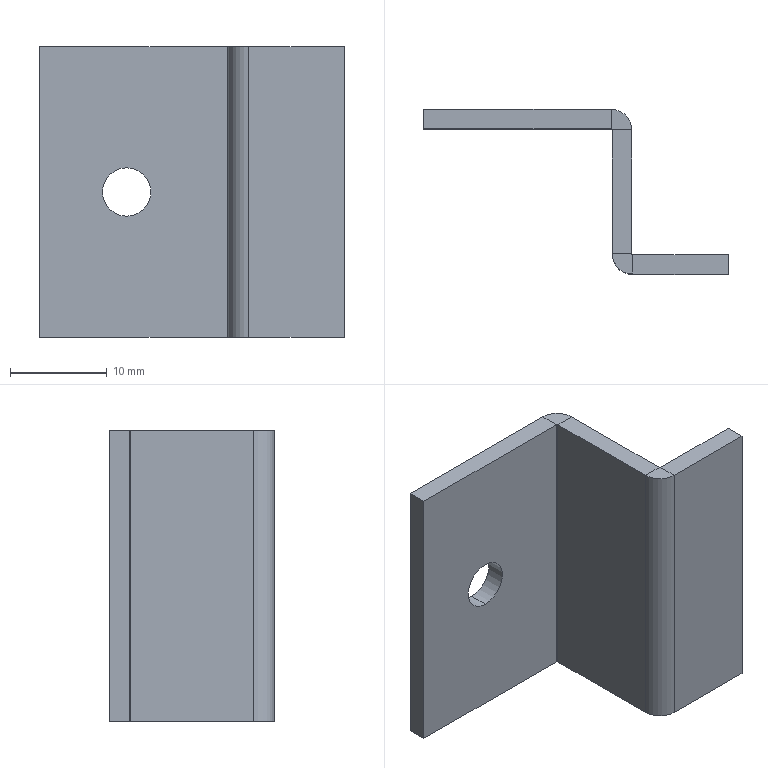Component | SolidWorks | FrontDoorAssembly-1_GlassRetainerPG50-02-105-10 | 1 solid | 24 faces | box 31.5 x 17 x 30 mm | volume 2694 mm3 | plane 18 | cylinder 6 | commonest cylinder face diameters 5 x2 4.2 x2 0.2 x2 | material AISI 1045 Steel, cold drawn
STEP:
#1=COLOUR_RGB('',0.7922,0.8196,0.9333);
#2=FILL_AREA_STYLE_COLOUR('',#1);
#3=FILL_AREA_STYLE('',(#2));
#4=SURFACE_STYLE_FILL_AREA(#3);
#5=SURFACE_SIDE_STYLE('',(#4));
#6=SURFACE_STYLE_USAGE(.BOTH.,#5);
#7=PRESENTATION_STYLE_ASSIGNMENT((#6));
#8=CARTESIAN_POINT('',(-43.629,-10.307,10.729));
#9=VERTEX_POINT('',#8);
#10=CARTESIAN_POINT('',(-43.629,-10.307,10.925));
#11=VERTEX_POINT('',#10);
#12=CARTESIAN_POINT('',(-43.629,-10.307,10.827));
#13=DIRECTION('',(-0.,1.,0.));
#14=DIRECTION('',(0.,0.,1.));
#15=AXIS2_PLACEMENT_3D('',#12,#13,#14);
#16=CIRCLE('',#15,0.09843);
#17=EDGE_CURVE('',#9,#11,#16,.T.);
#18=ORIENTED_EDGE('',*,*,#17,.F.);
#19=CARTESIAN_POINT('',(-43.629,-10.228,10.729));
#20=VERTEX_POINT('',#19);
#21=CARTESIAN_POINT('',(-43.629,-10.228,10.729));
#22=DIRECTION('',(-0.,1.,0.));
#23=VECTOR('',#22,39.37);
#24=LINE('',#21,#23);
#25=EDGE_CURVE('',#9,#20,#24,.T.);
#26=ORIENTED_EDGE('',*,*,#25,.T.);
#27=CARTESIAN_POINT('',(-43.629,-10.228,10.925));
#28=VERTEX_POINT('',#27);
#29=CARTESIAN_POINT('',(-43.629,-10.228,10.827));
#30=DIRECTION('',(-0.,1.,0.));
#31=DIRECTION('',(0.,0.,1.));
#32=AXIS2_PLACEMENT_3D('',#29,#30,#31);
#33=CIRCLE('',#32,0.09843);
#34=EDGE_CURVE('',#20,#28,#33,.T.);
#35=ORIENTED_EDGE('',*,*,#34,.T.);
#36=CARTESIAN_POINT('',(-43.629,-10.228,10.925));
#37=DIRECTION('',(-0.,1.,0.));
#38=VECTOR('',#37,39.37);
#39=LINE('',#36,#38);
#40=EDGE_CURVE('',#11,#28,#39,.T.);
#41=ORIENTED_EDGE('',*,*,#40,.F.);
#42=EDGE_LOOP('',(#18,#26,#35,#41));
#43=FACE_OUTER_BOUND('',#42,.T.);
#44=CARTESIAN_POINT('',(-43.629,-10.228,10.827));
#45=DIRECTION('',(-0.,1.,0.));
#46=DIRECTION('',(0.,0.,1.));
#47=AXIS2_PLACEMENT_3D('',#44,#45,#46);
#48=CYLINDRICAL_SURFACE('',#47,0.09843);
#49=ADVANCED_FACE('',(#43),#48,.F.);
#50=CARTESIAN_POINT('',(-43.216,-10.815,10.236));
#51=VERTEX_POINT('',#50);
#52=CARTESIAN_POINT('',(-43.137,-10.815,10.236));
#53=VERTEX_POINT('',#52);
#54=CARTESIAN_POINT('',(-43.137,-10.815,10.236));
#55=DIRECTION('',(1.,0.,0.));
#56=VECTOR('',#55,39.37);
#57=LINE('',#54,#56);
#58=EDGE_CURVE('',#51,#53,#57,.T.);
#59=ORIENTED_EDGE('',*,*,#58,.F.);
#60=CARTESIAN_POINT('',(-43.216,-10.311,10.236));
#61=VERTEX_POINT('',#60);
#62=CARTESIAN_POINT('',(-43.216,-10.819,10.236));
#63=DIRECTION('',(0.,-1.,-0.));
#64=VECTOR('',#63,39.37);
#65=LINE('',#62,#64);
#66=EDGE_CURVE('',#61,#51,#65,.T.);
#67=ORIENTED_EDGE('',*,*,#66,.F.);
#68=CARTESIAN_POINT('',(-43.137,-10.311,10.236));
#69=VERTEX_POINT('',#68);
#70=CARTESIAN_POINT('',(-43.137,-10.311,10.236));
#71=DIRECTION('',(1.,0.,0.));
#72=VECTOR('',#71,39.37);
#73=LINE('',#70,#72);
#74=EDGE_CURVE('',#61,#69,#73,.T.);
#75=ORIENTED_EDGE('',*,*,#74,.T.);
#76=CARTESIAN_POINT('',(-43.137,-10.819,10.236));
#77=DIRECTION('',(0.,-1.,-0.));
#78=VECTOR('',#77,39.37);
#79=LINE('',#76,#78);
#80=EDGE_CURVE('',#69,#53,#79,.T.);
#81=ORIENTED_EDGE('',*,*,#80,.T.);
#82=EDGE_LOOP('',(#59,#67,#75,#81));
#83=FACE_OUTER_BOUND('',#82,.T.);
#84=CARTESIAN_POINT('',(-43.137,-10.819,10.236));
#85=DIRECTION('',(0.,0.,-1.));
#86=DIRECTION('',(0.,-1.,-0.));
#87=AXIS2_PLACEMENT_3D('',#84,#85,#86);
#88=PLANE('',#87);
#89=ADVANCED_FACE('',(#83),#88,.T.);
#90=ORIENTED_EDGE('',*,*,#74,.F.);
#91=CARTESIAN_POINT('',(-43.22,-10.307,10.236));
#92=VERTEX_POINT('',#91);
#93=CARTESIAN_POINT('',(-43.22,-10.311,10.236));
#94=DIRECTION('',(-0.,-0.,1.));
#95=DIRECTION('',(0.,-1.,0.));
#96=AXIS2_PLACEMENT_3D('',#93,#94,#95);
#97=CIRCLE('',#96,0.003937);
#98=EDGE_CURVE('',#61,#92,#97,.T.);
#99=ORIENTED_EDGE('',*,*,#98,.T.);
#100=CARTESIAN_POINT('',(-43.22,-10.228,10.236));
#101=VERTEX_POINT('',#100);
#102=CARTESIAN_POINT('',(-43.22,-10.228,10.236));
#103=DIRECTION('',(-0.,1.,0.));
#104=VECTOR('',#103,39.37);
#105=LINE('',#102,#104);
#106=EDGE_CURVE('',#92,#101,#105,.T.);
#107=ORIENTED_EDGE('',*,*,#106,.T.);
#108=CARTESIAN_POINT('',(-43.22,-10.311,10.236));
#109=DIRECTION('',(-0.,-0.,1.));
#110=DIRECTION('',(0.,1.,0.));
#111=AXIS2_PLACEMENT_3D('',#108,#109,#110);
#112=CIRCLE('',#111,0.08268);
#113=EDGE_CURVE('',#69,#101,#112,.T.);
#114=ORIENTED_EDGE('',*,*,#113,.F.);
#115=EDGE_LOOP('',(#90,#99,#107,#114));
#116=FACE_OUTER_BOUND('',#115,.T.);
#117=CARTESIAN_POINT('',(-43.22,-10.311,10.236));
#118=DIRECTION('',(-0.,-0.,1.));
#119=DIRECTION('',(0.,-1.,-0.));
#120=AXIS2_PLACEMENT_3D('',#117,#118,#119);
#121=PLANE('',#120);
#122=ADVANCED_FACE('',(#116),#121,.F.);
#123=ORIENTED_EDGE('',*,*,#106,.F.);
#124=CARTESIAN_POINT('',(-43.984,-10.307,10.236));
#125=VERTEX_POINT('',#124);
#126=CARTESIAN_POINT('',(-43.137,-10.307,10.236));
#127=DIRECTION('',(1.,0.,0.));
#128=VECTOR('',#127,39.37);
#129=LINE('',#126,#128);
#130=EDGE_CURVE('',#125,#92,#129,.T.);
#131=ORIENTED_EDGE('',*,*,#130,.F.);
#132=CARTESIAN_POINT('',(-43.984,-10.228,10.236));
#133=VERTEX_POINT('',#132);
#134=CARTESIAN_POINT('',(-43.984,-10.228,10.236));
#135=DIRECTION('',(-0.,1.,0.));
#136=VECTOR('',#135,39.37);
#137=LINE('',#134,#136);
#138=EDGE_CURVE('',#125,#133,#137,.T.);
#139=ORIENTED_EDGE('',*,*,#138,.T.);
#140=CARTESIAN_POINT('',(-43.137,-10.228,10.236));
#141=DIRECTION('',(1.,0.,0.));
#142=VECTOR('',#141,39.37);
#143=LINE('',#140,#142);
#144=EDGE_CURVE('',#133,#101,#143,.T.);
#145=ORIENTED_EDGE('',*,*,#144,.T.);
#146=EDGE_LOOP('',(#123,#131,#139,#145));
#147=FACE_OUTER_BOUND('',#146,.T.);
#148=CARTESIAN_POINT('',(-43.137,-10.228,10.236));
#149=DIRECTION('',(0.,0.,-1.));
#150=DIRECTION('',(1.,0.,0.));
#151=AXIS2_PLACEMENT_3D('',#148,#149,#150);
#152=PLANE('',#151);
#153=ADVANCED_FACE('',(#147),#152,.T.);
#154=ORIENTED_EDGE('',*,*,#138,.F.);
#155=CARTESIAN_POINT('',(-43.984,-10.307,11.417));
#156=VERTEX_POINT('',#155);
#157=CARTESIAN_POINT('',(-43.984,-10.307,10.236));
#158=DIRECTION('',(-0.,-0.,1.));
#159=VECTOR('',#158,39.37);
#160=LINE('',#157,#159);
#161=EDGE_CURVE('',#125,#156,#160,.T.);
#162=ORIENTED_EDGE('',*,*,#161,.T.);
#163=CARTESIAN_POINT('',(-43.984,-10.228,11.417));
#164=VERTEX_POINT('',#163);
#165=CARTESIAN_POINT('',(-43.984,-10.228,11.417));
#166=DIRECTION('',(-0.,1.,0.));
#167=VECTOR('',#166,39.37);
#168=LINE('',#165,#167);
#169=EDGE_CURVE('',#156,#164,#168,.T.);
#170=ORIENTED_EDGE('',*,*,#169,.T.);
#171=CARTESIAN_POINT('',(-43.984,-10.228,10.236));
#172=DIRECTION('',(-0.,-0.,1.));
#173=VECTOR('',#172,39.37);
#174=LINE('',#171,#173);
#175=EDGE_CURVE('',#133,#164,#174,.T.);
#176=ORIENTED_EDGE('',*,*,#175,.F.);
#177=EDGE_LOOP('',(#154,#162,#170,#176));
#178=FACE_OUTER_BOUND('',#177,.T.);
#179=CARTESIAN_POINT('',(-43.984,-10.228,10.236));
#180=DIRECTION('',(1.,0.,0.));
#181=DIRECTION('',(-0.,-0.,1.));
#182=AXIS2_PLACEMENT_3D('',#179,#180,#181);
#183=PLANE('',#182);
#184=ADVANCED_FACE('',(#178),#183,.F.);
#185=ORIENTED_EDGE('',*,*,#169,.F.);
#186=CARTESIAN_POINT('',(-43.22,-10.307,11.417));
#187=VERTEX_POINT('',#186);
#188=CARTESIAN_POINT('',(-43.137,-10.307,11.417));
#189=DIRECTION('',(1.,0.,0.));
#190=VECTOR('',#189,39.37);
#191=LINE('',#188,#190);
#192=EDGE_CURVE('',#156,#187,#191,.T.);
#193=ORIENTED_EDGE('',*,*,#192,.T.);
#194=CARTESIAN_POINT('',(-43.22,-10.228,11.417));
#195=VERTEX_POINT('',#194);
#196=CARTESIAN_POINT('',(-43.22,-10.228,11.417));
#197=DIRECTION('',(-0.,1.,0.));
#198=VECTOR('',#197,39.37);
#199=LINE('',#196,#198);
#200=EDGE_CURVE('',#187,#195,#199,.T.);
#201=ORIENTED_EDGE('',*,*,#200,.T.);
#202=CARTESIAN_POINT('',(-43.137,-10.228,11.417));
#203=DIRECTION('',(1.,0.,0.));
#204=VECTOR('',#203,39.37);
#205=LINE('',#202,#204);
#206=EDGE_CURVE('',#164,#195,#205,.T.);
#207=ORIENTED_EDGE('',*,*,#206,.F.);
#208=EDGE_LOOP('',(#185,#193,#201,#207));
#209=FACE_OUTER_BOUND('',#208,.T.);
#210=CARTESIAN_POINT('',(-43.137,-10.228,11.417));
#211=DIRECTION('',(0.,0.,-1.));
#212=DIRECTION('',(1.,0.,0.));
#213=AXIS2_PLACEMENT_3D('',#210,#211,#212);
#214=PLANE('',#213);
#215=ADVANCED_FACE('',(#209),#214,.F.);
#216=ORIENTED_EDGE('',*,*,#200,.F.);
#217=CARTESIAN_POINT('',(-43.216,-10.311,11.417));
#218=VERTEX_POINT('',#217);
#219=CARTESIAN_POINT('',(-43.22,-10.311,11.417));
#220=DIRECTION('',(0.,0.,-1.));
#221=DIRECTION('',(0.,-1.,0.));
#222=AXIS2_PLACEMENT_3D('',#219,#220,#221);
#223=CIRCLE('',#222,0.003937);
#224=EDGE_CURVE('',#187,#218,#223,.T.);
#225=ORIENTED_EDGE('',*,*,#224,.T.);
#226=CARTESIAN_POINT('',(-43.137,-10.311,11.417));
#227=VERTEX_POINT('',#226);
#228=CARTESIAN_POINT('',(-43.137,-10.311,11.417));
#229=DIRECTION('',(1.,0.,0.));
#230=VECTOR('',#229,39.37);
#231=LINE('',#228,#230);
#232=EDGE_CURVE('',#218,#227,#231,.T.);
#233=ORIENTED_EDGE('',*,*,#232,.T.);
#234=CARTESIAN_POINT('',(-43.22,-10.311,11.417));
#235=DIRECTION('',(0.,0.,-1.));
#236=DIRECTION('',(0.,-1.,0.));
#237=AXIS2_PLACEMENT_3D('',#234,#235,#236);
#238=CIRCLE('',#237,0.08268);
#239=EDGE_CURVE('',#195,#227,#238,.T.);
#240=ORIENTED_EDGE('',*,*,#239,.F.);
#241=EDGE_LOOP('',(#216,#225,#233,#240));
#242=FACE_OUTER_BOUND('',#241,.T.);
#243=CARTESIAN_POINT('',(-43.22,-10.311,11.417));
#244=DIRECTION('',(0.,0.,-1.));
#245=DIRECTION('',(-0.,1.,0.));
#246=AXIS2_PLACEMENT_3D('',#243,#244,#245);
#247=PLANE('',#246);
#248=ADVANCED_FACE('',(#242),#247,.F.);
#249=ORIENTED_EDGE('',*,*,#232,.F.);
#250=CARTESIAN_POINT('',(-43.216,-10.815,11.417));
#251=VERTEX_POINT('',#250);
#252=CARTESIAN_POINT('',(-43.216,-10.819,11.417));
#253=DIRECTION('',(0.,-1.,-0.));
#254=VECTOR('',#253,39.37);
#255=LINE('',#252,#254);
#256=EDGE_CURVE('',#218,#251,#255,.T.);
#257=ORIENTED_EDGE('',*,*,#256,.T.);
#258=CARTESIAN_POINT('',(-43.137,-10.815,11.417));
#259=VERTEX_POINT('',#258);
#260=CARTESIAN_POINT('',(-43.137,-10.815,11.417));
#261=DIRECTION('',(1.,0.,0.));
#262=VECTOR('',#261,39.37);
#263=LINE('',#260,#262);
#264=EDGE_CURVE('',#251,#259,#263,.T.);
#265=ORIENTED_EDGE('',*,*,#264,.T.);
#266=CARTESIAN_POINT('',(-43.137,-10.819,11.417));
#267=DIRECTION('',(0.,-1.,-0.));
#268=VECTOR('',#267,39.37);
#269=LINE('',#266,#268);
#270=EDGE_CURVE('',#227,#259,#269,.T.);
#271=ORIENTED_EDGE('',*,*,#270,.F.);
#272=EDGE_LOOP('',(#249,#257,#265,#271));
#273=FACE_OUTER_BOUND('',#272,.T.);
#274=CARTESIAN_POINT('',(-43.137,-10.819,11.417));
#275=DIRECTION('',(0.,0.,-1.));
#276=DIRECTION('',(0.,-1.,-0.));
#277=AXIS2_PLACEMENT_3D('',#274,#275,#276);
#278=PLANE('',#277);
#279=ADVANCED_FACE('',(#273),#278,.F.);
#280=ORIENTED_EDGE('',*,*,#264,.F.);
#281=CARTESIAN_POINT('',(-43.133,-10.898,11.417));
#282=VERTEX_POINT('',#281);
#283=CARTESIAN_POINT('',(-43.133,-10.815,11.417));
#284=DIRECTION('',(-0.,-0.,1.));
#285=DIRECTION('',(0.,1.,0.));
#286=AXIS2_PLACEMENT_3D('',#283,#284,#285);
#287=CIRCLE('',#286,0.08268);
#288=EDGE_CURVE('',#251,#282,#287,.T.);
#289=ORIENTED_EDGE('',*,*,#288,.T.);
#290=CARTESIAN_POINT('',(-43.133,-10.819,11.417));
#291=VERTEX_POINT('',#290);
#292=CARTESIAN_POINT('',(-43.133,-10.819,11.417));
#293=DIRECTION('',(-0.,1.,0.));
#294=VECTOR('',#293,39.37);
#295=LINE('',#292,#294);
#296=EDGE_CURVE('',#282,#291,#295,.T.);
#297=ORIENTED_EDGE('',*,*,#296,.T.);
#298=CARTESIAN_POINT('',(-43.133,-10.815,11.417));
#299=DIRECTION('',(-0.,-0.,1.));
#300=DIRECTION('',(0.,1.,0.));
#301=AXIS2_PLACEMENT_3D('',#298,#299,#300);
#302=CIRCLE('',#301,0.003937);
#303=EDGE_CURVE('',#259,#291,#302,.T.);
#304=ORIENTED_EDGE('',*,*,#303,.F.);
#305=EDGE_LOOP('',(#280,#289,#297,#304));
#306=FACE_OUTER_BOUND('',#305,.T.);
#307=CARTESIAN_POINT('',(-43.133,-10.815,11.417));
#308=DIRECTION('',(-0.,-0.,1.));
#309=DIRECTION('',(0.,-1.,-0.));
#310=AXIS2_PLACEMENT_3D('',#307,#308,#309);
#311=PLANE('',#310);
#312=ADVANCED_FACE('',(#306),#311,.T.);
#313=CARTESIAN_POINT('',(-42.744,-10.898,11.417));
#314=VERTEX_POINT('',#313);
#315=CARTESIAN_POINT('',(-42.744,-10.819,11.417));
#316=VERTEX_POINT('',#315);
#317=CARTESIAN_POINT('',(-42.744,-11.213,11.417));
#318=DIRECTION('',(-0.,1.,0.));
#319=VECTOR('',#318,39.37);
#320=LINE('',#317,#319);
#321=EDGE_CURVE('',#314,#316,#320,.T.);
#322=ORIENTED_EDGE('',*,*,#321,.T.);
#323=CARTESIAN_POINT('',(-42.629,-10.819,11.417));
#324=DIRECTION('',(1.,0.,0.));
#325=VECTOR('',#324,39.37);
#326=LINE('',#323,#325);
#327=EDGE_CURVE('',#291,#316,#326,.T.);
#328=ORIENTED_EDGE('',*,*,#327,.F.);
#329=ORIENTED_EDGE('',*,*,#296,.F.);
#330=CARTESIAN_POINT('',(-42.629,-10.898,11.417));
#331=DIRECTION('',(1.,0.,0.));
#332=VECTOR('',#331,39.37);
#333=LINE('',#330,#332);
#334=EDGE_CURVE('',#282,#314,#333,.T.);
#335=ORIENTED_EDGE('',*,*,#334,.T.);
#336=EDGE_LOOP('',(#322,#328,#329,#335));
#337=FACE_OUTER_BOUND('',#336,.T.);
#338=CARTESIAN_POINT('',(-42.629,-10.819,11.417));
#339=DIRECTION('',(0.,0.,-1.));
#340=DIRECTION('',(1.,0.,0.));
#341=AXIS2_PLACEMENT_3D('',#338,#339,#340);
#342=PLANE('',#341);
#343=ADVANCED_FACE('',(#337),#342,.F.);
#344=CARTESIAN_POINT('',(-42.744,-10.898,10.236));
#345=VERTEX_POINT('',#344);
#346=CARTESIAN_POINT('',(-42.744,-10.819,10.236));
#347=VERTEX_POINT('',#346);
#348=CARTESIAN_POINT('',(-42.744,-11.213,10.236));
#349=DIRECTION('',(-0.,1.,0.));
#350=VECTOR('',#349,39.37);
#351=LINE('',#348,#350);
#352=EDGE_CURVE('',#345,#347,#351,.T.);
#353=ORIENTED_EDGE('',*,*,#352,.F.);
#354=CARTESIAN_POINT('',(-43.133,-10.898,10.236));
#355=VERTEX_POINT('',#354);
#356=CARTESIAN_POINT('',(-42.629,-10.898,10.236));
#357=DIRECTION('',(1.,0.,0.));
#358=VECTOR('',#357,39.37);
#359=LINE('',#356,#358);
#360=EDGE_CURVE('',#355,#345,#359,.T.);
#361=ORIENTED_EDGE('',*,*,#360,.F.);
#362=CARTESIAN_POINT('',(-43.133,-10.819,10.236));
#363=VERTEX_POINT('',#362);
#364=CARTESIAN_POINT('',(-43.133,-10.819,10.236));
#365=DIRECTION('',(-0.,1.,0.));
#366=VECTOR('',#365,39.37);
#367=LINE('',#364,#366);
#368=EDGE_CURVE('',#355,#363,#367,.T.);
#369=ORIENTED_EDGE('',*,*,#368,.T.);
#370=CARTESIAN_POINT('',(-42.629,-10.819,10.236));
#371=DIRECTION('',(1.,0.,0.));
#372=VECTOR('',#371,39.37);
#373=LINE('',#370,#372);
#374=EDGE_CURVE('',#363,#347,#373,.T.);
#375=ORIENTED_EDGE('',*,*,#374,.T.);
#376=EDGE_LOOP('',(#353,#361,#369,#375));
#377=FACE_OUTER_BOUND('',#376,.T.);
#378=CARTESIAN_POINT('',(-42.629,-10.819,10.236));
#379=DIRECTION('',(0.,0.,-1.));
#380=DIRECTION('',(1.,0.,0.));
#381=AXIS2_PLACEMENT_3D('',#378,#379,#380);
#382=PLANE('',#381);
#383=ADVANCED_FACE('',(#377),#382,.T.);
#384=ORIENTED_EDGE('',*,*,#25,.F.);
#385=CARTESIAN_POINT('',(-43.629,-10.307,10.827));
#386=DIRECTION('',(-0.,1.,0.));
#387=DIRECTION('',(0.,0.,1.));
#388=AXIS2_PLACEMENT_3D('',#385,#386,#387);
#389=CIRCLE('',#388,0.09843);
#390=EDGE_CURVE('',#11,#9,#389,.T.);
#391=ORIENTED_EDGE('',*,*,#390,.F.);
#392=ORIENTED_EDGE('',*,*,#40,.T.);
#393=CARTESIAN_POINT('',(-43.629,-10.228,10.827));
#394=DIRECTION('',(-0.,1.,0.));
#395=DIRECTION('',(0.,0.,1.));
#396=AXIS2_PLACEMENT_3D('',#393,#394,#395);
#397=CIRCLE('',#396,0.09843);
#398=EDGE_CURVE('',#28,#20,#397,.T.);
#399=ORIENTED_EDGE('',*,*,#398,.T.);
#400=EDGE_LOOP('',(#384,#391,#392,#399));
#401=FACE_OUTER_BOUND('',#400,.T.);
#402=CARTESIAN_POINT('',(-43.629,-10.228,10.827));
#403=DIRECTION('',(-0.,1.,0.));
#404=DIRECTION('',(0.,0.,1.));
#405=AXIS2_PLACEMENT_3D('',#402,#403,#404);
#406=CYLINDRICAL_SURFACE('',#405,0.09843);
#407=ADVANCED_FACE('',(#401),#406,.F.);
#408=CARTESIAN_POINT('',(-43.133,-10.815,10.236));
#409=DIRECTION('',(0.,0.,-1.));
#410=DIRECTION('',(0.,1.,0.));
#411=AXIS2_PLACEMENT_3D('',#408,#409,#410);
#412=CIRCLE('',#411,0.08268);
#413=EDGE_CURVE('',#355,#51,#412,.T.);
#414=ORIENTED_EDGE('',*,*,#413,.T.);
#415=ORIENTED_EDGE('',*,*,#58,.T.);
#416=CARTESIAN_POINT('',(-43.133,-10.815,10.236));
#417=DIRECTION('',(0.,0.,-1.));
#418=DIRECTION('',(0.,-1.,0.));
#419=AXIS2_PLACEMENT_3D('',#416,#417,#418);
#420=CIRCLE('',#419,0.003937);
#421=EDGE_CURVE('',#363,#53,#420,.T.);
#422=ORIENTED_EDGE('',*,*,#421,.F.);
#423=ORIENTED_EDGE('',*,*,#368,.F.);
#424=EDGE_LOOP('',(#414,#415,#422,#423));
#425=FACE_OUTER_BOUND('',#424,.T.);
#426=CARTESIAN_POINT('',(-43.133,-10.815,10.236));
#427=DIRECTION('',(0.,0.,-1.));
#428=DIRECTION('',(-0.,1.,0.));
#429=AXIS2_PLACEMENT_3D('',#426,#427,#428);
#430=PLANE('',#429);
#431=ADVANCED_FACE('',(#425),#430,.T.);
#432=ORIENTED_EDGE('',*,*,#327,.T.);
#433=CARTESIAN_POINT('',(-42.744,-10.819,10.236));
#434=DIRECTION('',(-0.,-0.,1.));
#435=VECTOR('',#434,39.37);
#436=LINE('',#433,#435);
#437=EDGE_CURVE('',#347,#316,#436,.T.);
#438=ORIENTED_EDGE('',*,*,#437,.F.);
#439=ORIENTED_EDGE('',*,*,#374,.F.);
#440=CARTESIAN_POINT('',(-43.133,-10.819,11.417));
#441=DIRECTION('',(-0.,-0.,1.));
#442=VECTOR('',#441,39.37);
#443=LINE('',#440,#442);
#444=EDGE_CURVE('',#363,#291,#443,.T.);
#445=ORIENTED_EDGE('',*,*,#444,.T.);
#446=EDGE_LOOP('',(#432,#438,#439,#445));
#447=FACE_OUTER_BOUND('',#446,.T.);
#448=CARTESIAN_POINT('',(-42.629,-10.819,10.236));
#449=DIRECTION('',(0.,-1.,-0.));
#450=DIRECTION('',(0.,0.,-1.));
#451=AXIS2_PLACEMENT_3D('',#448,#449,#450);
#452=PLANE('',#451);
#453=ADVANCED_FACE('',(#447),#452,.F.);
#454=ORIENTED_EDGE('',*,*,#398,.F.);
#455=ORIENTED_EDGE('',*,*,#34,.F.);
#456=EDGE_LOOP('',(#454,#455));
#457=FACE_BOUND('',#456,.T.);
#458=ORIENTED_EDGE('',*,*,#206,.T.);
#459=CARTESIAN_POINT('',(-43.22,-10.228,10.236));
#460=DIRECTION('',(0.,0.,-1.));
#461=VECTOR('',#460,39.37);
#462=LINE('',#459,#461);
#463=EDGE_CURVE('',#195,#101,#462,.T.);
#464=ORIENTED_EDGE('',*,*,#463,.T.);
#465=ORIENTED_EDGE('',*,*,#144,.F.);
#466=ORIENTED_EDGE('',*,*,#175,.T.);
#467=EDGE_LOOP('',(#458,#464,#465,#466));
#468=FACE_OUTER_BOUND('',#467,.T.);
#469=CARTESIAN_POINT('',(-43.137,-10.228,10.236));
#470=DIRECTION('',(0.,-1.,-0.));
#471=DIRECTION('',(0.,0.,-1.));
#472=AXIS2_PLACEMENT_3D('',#469,#470,#471);
#473=PLANE('',#472);
#474=ADVANCED_FACE('',(#457,#468),#473,.F.);
#475=ORIENTED_EDGE('',*,*,#270,.T.);
#476=CARTESIAN_POINT('',(-43.137,-10.815,10.236));
#477=DIRECTION('',(0.,0.,-1.));
#478=VECTOR('',#477,39.37);
#479=LINE('',#476,#478);
#480=EDGE_CURVE('',#259,#53,#479,.T.);
#481=ORIENTED_EDGE('',*,*,#480,.T.);
#482=ORIENTED_EDGE('',*,*,#80,.F.);
#483=CARTESIAN_POINT('',(-43.137,-10.311,10.236));
#484=DIRECTION('',(-0.,-0.,1.));
#485=VECTOR('',#484,39.37);
#486=LINE('',#483,#485);
#487=EDGE_CURVE('',#69,#227,#486,.T.);
#488=ORIENTED_EDGE('',*,*,#487,.T.);
#489=EDGE_LOOP('',(#475,#481,#482,#488));
#490=FACE_OUTER_BOUND('',#489,.T.);
#491=CARTESIAN_POINT('',(-43.137,-10.819,10.236));
#492=DIRECTION('',(-1.,-0.,-0.));
#493=DIRECTION('',(-0.,1.,0.));
#494=AXIS2_PLACEMENT_3D('',#491,#492,#493);
#495=PLANE('',#494);
#496=ADVANCED_FACE('',(#490),#495,.F.);
#497=ORIENTED_EDGE('',*,*,#113,.T.);
#498=ORIENTED_EDGE('',*,*,#463,.F.);
#499=ORIENTED_EDGE('',*,*,#239,.T.);
#500=ORIENTED_EDGE('',*,*,#487,.F.);
#501=EDGE_LOOP('',(#497,#498,#499,#500));
#502=FACE_OUTER_BOUND('',#501,.T.);
#503=CARTESIAN_POINT('',(-43.22,-10.311,10.236));
#504=DIRECTION('',(-0.,-0.,1.));
#505=DIRECTION('',(0.,-1.,0.));
#506=AXIS2_PLACEMENT_3D('',#503,#504,#505);
#507=CYLINDRICAL_SURFACE('',#506,0.08268);
#508=ADVANCED_FACE('',(#502),#507,.T.);
#509=ORIENTED_EDGE('',*,*,#421,.T.);
#510=ORIENTED_EDGE('',*,*,#480,.F.);
#511=ORIENTED_EDGE('',*,*,#303,.T.);
#512=ORIENTED_EDGE('',*,*,#444,.F.);
#513=EDGE_LOOP('',(#509,#510,#511,#512));
#514=FACE_OUTER_BOUND('',#513,.T.);
#515=CARTESIAN_POINT('',(-43.133,-10.815,10.236));
#516=DIRECTION('',(0.,0.,-1.));
#517=DIRECTION('',(0.,1.,0.));
#518=AXIS2_PLACEMENT_3D('',#515,#516,#517);
#519=CYLINDRICAL_SURFACE('',#518,0.003937);
#520=ADVANCED_FACE('',(#514),#519,.F.);
#521=CARTESIAN_POINT('',(-42.744,-10.898,10.236));
#522=DIRECTION('',(0.,0.,-1.));
#523=VECTOR('',#522,39.37);
#524=LINE('',#521,#523);
#525=EDGE_CURVE('',#314,#345,#524,.T.);
#526=ORIENTED_EDGE('',*,*,#525,.F.);
#527=ORIENTED_EDGE('',*,*,#334,.F.);
#528=CARTESIAN_POINT('',(-43.133,-10.898,10.236));
#529=DIRECTION('',(-0.,-0.,1.));
#530=VECTOR('',#529,39.37);
#531=LINE('',#528,#530);
#532=EDGE_CURVE('',#355,#282,#531,.T.);
#533=ORIENTED_EDGE('',*,*,#532,.F.);
#534=ORIENTED_EDGE('',*,*,#360,.T.);
#535=EDGE_LOOP('',(#526,#527,#533,#534));
#536=FACE_OUTER_BOUND('',#535,.T.);
#537=CARTESIAN_POINT('',(-42.629,-10.898,10.236));
#538=DIRECTION('',(0.,-1.,-0.));
#539=DIRECTION('',(0.,0.,-1.));
#540=AXIS2_PLACEMENT_3D('',#537,#538,#539);
#541=PLANE('',#540);
#542=ADVANCED_FACE('',(#536),#541,.T.);
#543=ORIENTED_EDGE('',*,*,#390,.T.);
#544=ORIENTED_EDGE('',*,*,#17,.T.);
#545=EDGE_LOOP('',(#543,#544));
#546=FACE_BOUND('',#545,.T.);
#547=ORIENTED_EDGE('',*,*,#192,.F.);
#548=ORIENTED_EDGE('',*,*,#161,.F.);
#549=ORIENTED_EDGE('',*,*,#130,.T.);
#550=CARTESIAN_POINT('',(-43.22,-10.307,10.236));
#551=DIRECTION('',(0.,0.,-1.));
#552=VECTOR('',#551,39.37);
#553=LINE('',#550,#552);
#554=EDGE_CURVE('',#187,#92,#553,.T.);
#555=ORIENTED_EDGE('',*,*,#554,.F.);
#556=EDGE_LOOP('',(#547,#548,#549,#555));
#557=FACE_OUTER_BOUND('',#556,.T.);
#558=CARTESIAN_POINT('',(-43.137,-10.307,10.236));
#559=DIRECTION('',(0.,-1.,-0.));
#560=DIRECTION('',(0.,0.,-1.));
#561=AXIS2_PLACEMENT_3D('',#558,#559,#560);
#562=PLANE('',#561);
#563=ADVANCED_FACE('',(#546,#557),#562,.T.);
#564=ORIENTED_EDGE('',*,*,#256,.F.);
#565=CARTESIAN_POINT('',(-43.216,-10.311,10.236));
#566=DIRECTION('',(-0.,-0.,1.));
#567=VECTOR('',#566,39.37);
#568=LINE('',#565,#567);
#569=EDGE_CURVE('',#61,#218,#568,.T.);
#570=ORIENTED_EDGE('',*,*,#569,.F.);
#571=ORIENTED_EDGE('',*,*,#66,.T.);
#572=CARTESIAN_POINT('',(-43.216,-10.815,10.236));
#573=DIRECTION('',(0.,0.,-1.));
#574=VECTOR('',#573,39.37);
#575=LINE('',#572,#574);
#576=EDGE_CURVE('',#251,#51,#575,.T.);
#577=ORIENTED_EDGE('',*,*,#576,.F.);
#578=EDGE_LOOP('',(#564,#570,#571,#577));
#579=FACE_OUTER_BOUND('',#578,.T.);
#580=CARTESIAN_POINT('',(-43.216,-10.819,10.236));
#581=DIRECTION('',(-1.,-0.,-0.));
#582=DIRECTION('',(-0.,1.,0.));
#583=AXIS2_PLACEMENT_3D('',#580,#581,#582);
#584=PLANE('',#583);
#585=ADVANCED_FACE('',(#579),#584,.T.);
#586=ORIENTED_EDGE('',*,*,#98,.F.);
#587=ORIENTED_EDGE('',*,*,#569,.T.);
#588=ORIENTED_EDGE('',*,*,#224,.F.);
#589=ORIENTED_EDGE('',*,*,#554,.T.);
#590=EDGE_LOOP('',(#586,#587,#588,#589));
#591=FACE_OUTER_BOUND('',#590,.T.);
#592=CARTESIAN_POINT('',(-43.22,-10.311,10.236));
#593=DIRECTION('',(-0.,-0.,1.));
#594=DIRECTION('',(0.,-1.,0.));
#595=AXIS2_PLACEMENT_3D('',#592,#593,#594);
#596=CYLINDRICAL_SURFACE('',#595,0.003937);
#597=ADVANCED_FACE('',(#591),#596,.F.);
#598=ORIENTED_EDGE('',*,*,#413,.F.);
#599=ORIENTED_EDGE('',*,*,#532,.T.);
#600=ORIENTED_EDGE('',*,*,#288,.F.);
#601=ORIENTED_EDGE('',*,*,#576,.T.);
#602=EDGE_LOOP('',(#598,#599,#600,#601));
#603=FACE_OUTER_BOUND('',#602,.T.);
#604=CARTESIAN_POINT('',(-43.133,-10.815,10.236));
#605=DIRECTION('',(0.,0.,-1.));
#606=DIRECTION('',(0.,1.,0.));
#607=AXIS2_PLACEMENT_3D('',#604,#605,#606);
#608=CYLINDRICAL_SURFACE('',#607,0.08268);
#609=ADVANCED_FACE('',(#603),#608,.T.);
#610=ORIENTED_EDGE('',*,*,#525,.T.);
#611=ORIENTED_EDGE('',*,*,#352,.T.);
#612=ORIENTED_EDGE('',*,*,#437,.T.);
#613=ORIENTED_EDGE('',*,*,#321,.F.);
#614=EDGE_LOOP('',(#610,#611,#612,#613));
#615=FACE_OUTER_BOUND('',#614,.T.);
#616=CARTESIAN_POINT('',(-42.744,-11.213,10.236));
#617=DIRECTION('',(-1.,-0.,-0.));
#618=DIRECTION('',(-0.,1.,0.));
#619=AXIS2_PLACEMENT_3D('',#616,#617,#618);
#620=PLANE('',#619);
#621=ADVANCED_FACE('',(#615),#620,.F.);
#622=CLOSED_SHELL('',(#49,#89,#122,#153,#184,#215,#248,#279,#312,#343,#383,#407,#431,#453,#474,#496,#508,#520,#542,#563,#585,#597,#609,#621));
#623=MANIFOLD_SOLID_BREP('',#622);
#624=STYLED_ITEM('',(#7),#623);
#625=PRESENTATION_LAYER_ASSIGNMENT('','',(#624));
#626=(LENGTH_UNIT()NAMED_UNIT(*)SI_UNIT($,.METRE.));
#627=LENGTH_MEASURE_WITH_UNIT(LENGTH_MEASURE(0.0254),#626);
#628=DIMENSIONAL_EXPONENTS(1.,0.,0.,0.,0.,0.,0.);
#629=(CONVERSION_BASED_UNIT('',#627)LENGTH_UNIT()NAMED_UNIT(#628));
#630=UNCERTAINTY_MEASURE_WITH_UNIT(LENGTH_MEASURE(0.00001),#629,'','');
#631=(NAMED_UNIT(*)PLANE_ANGLE_UNIT()SI_UNIT($,.RADIAN.));
#632=(NAMED_UNIT(*)SI_UNIT($,.STERADIAN.)SOLID_ANGLE_UNIT());
#633=(GEOMETRIC_REPRESENTATION_CONTEXT(3)GLOBAL_UNCERTAINTY_ASSIGNED_CONTEXT((#630))GLOBAL_UNIT_ASSIGNED_CONTEXT((#629,#631,#632))REPRESENTATION_CONTEXT('',''));
#634=MECHANICAL_DESIGN_GEOMETRIC_PRESENTATION_REPRESENTATION('',(#624),#633);
#635=CARTESIAN_POINT('',(0.,0.,0.));
#636=DIRECTION('',(0.,0.,1.));
#637=DIRECTION('',(1.,0.,0.));
#638=AXIS2_PLACEMENT_3D('',#635,#636,#637);
#639=(LENGTH_UNIT()NAMED_UNIT(*)SI_UNIT($,.METRE.));
#640=LENGTH_MEASURE_WITH_UNIT(LENGTH_MEASURE(0.0254),#639);
#641=DIMENSIONAL_EXPONENTS(1.,0.,0.,0.,0.,0.,0.);
#642=(CONVERSION_BASED_UNIT('',#640)LENGTH_UNIT()NAMED_UNIT(#641));
#643=UNCERTAINTY_MEASURE_WITH_UNIT(LENGTH_MEASURE(0.00001),#642,'','');
#644=(NAMED_UNIT(*)PLANE_ANGLE_UNIT()SI_UNIT($,.RADIAN.));
#645=(NAMED_UNIT(*)SI_UNIT($,.STERADIAN.)SOLID_ANGLE_UNIT());
#646=(GEOMETRIC_REPRESENTATION_CONTEXT(3)GLOBAL_UNCERTAINTY_ASSIGNED_CONTEXT((#643))GLOBAL_UNIT_ASSIGNED_CONTEXT((#642,#644,#645))REPRESENTATION_CONTEXT('',''));
#647=ADVANCED_BREP_SHAPE_REPRESENTATION('',(#623,#638),#646);